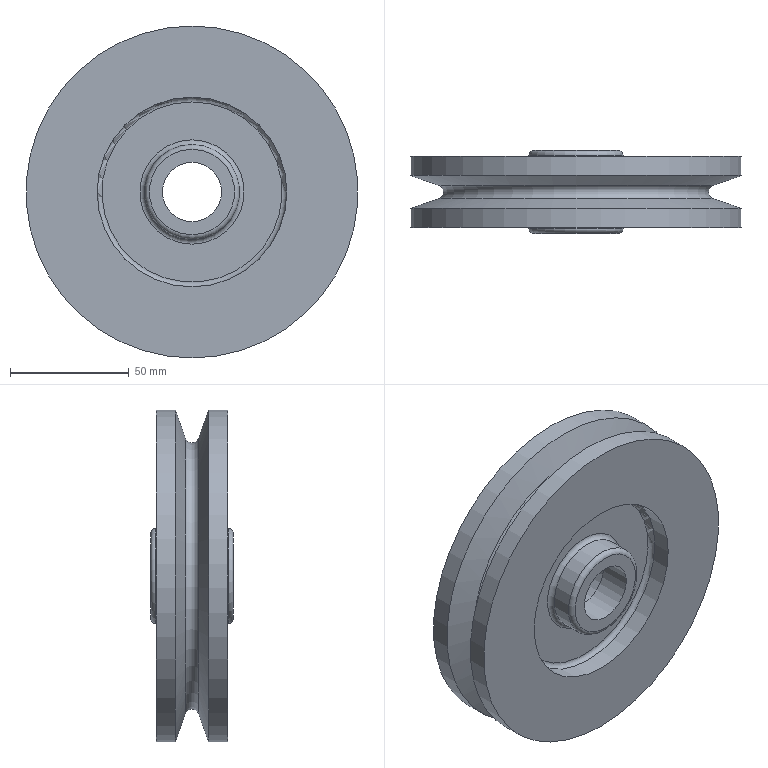Component | NX | 4 | 1 solid | 26 faces | volume 324017 mm3 | cylinder 9 | plane 8 | torus 7 | cone 2 | commonest cylinder face diameters 25 x2 40 x2 80 x2 140 x2 29 x1